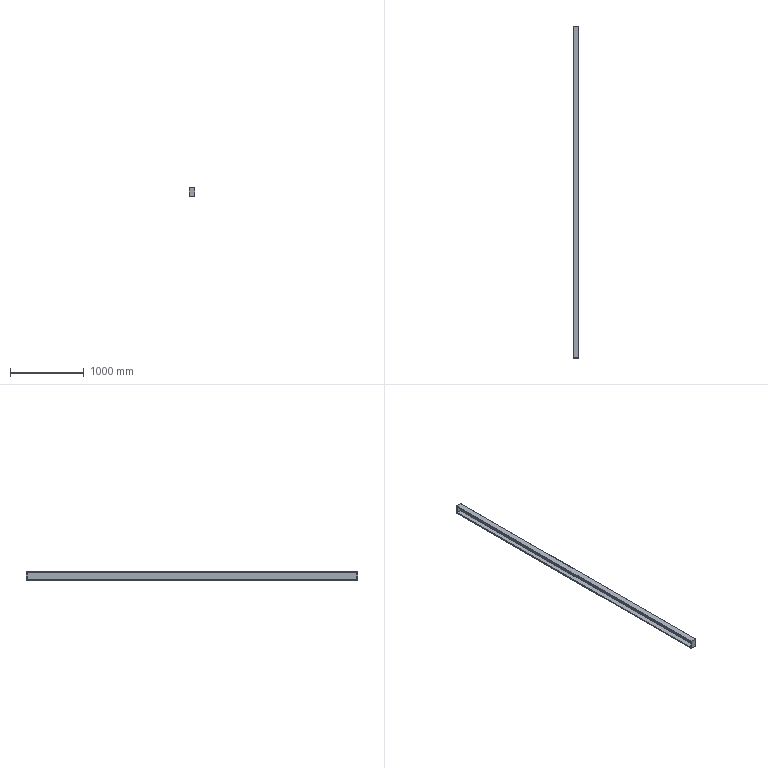Component | NX | CB9LIANJIE | 1 solid | 16 faces | volume 2083077 mm3 | plane 16